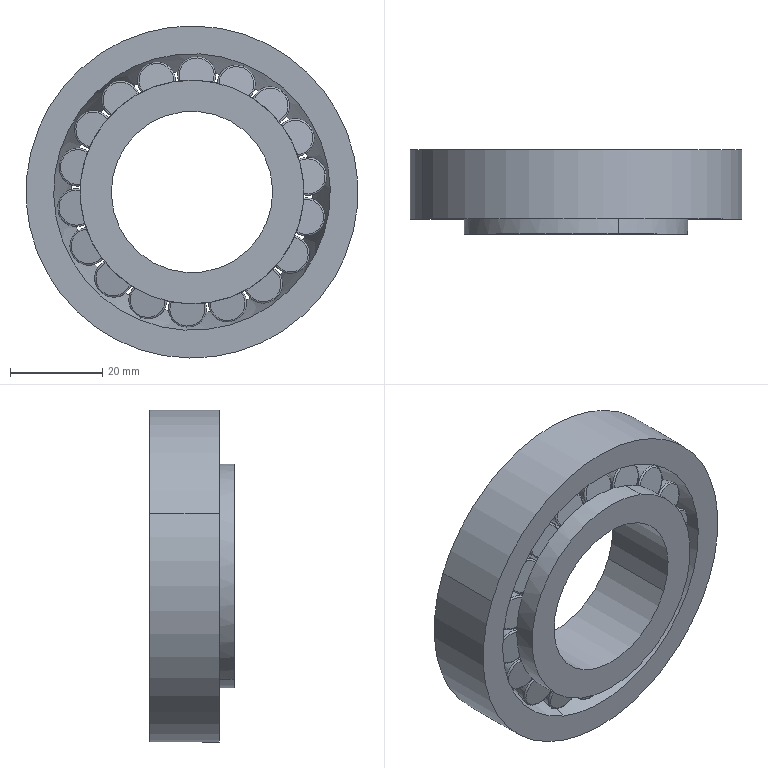Component | SolidWorks | 12-1 | 1 solid | 164 faces | volume 41399 mm3 | torus 72 | cone 44 | plane 40 | cylinder 8 | commonest cylinder face diameters 72 x2 35 x2 44.025 x2 48.5 x2